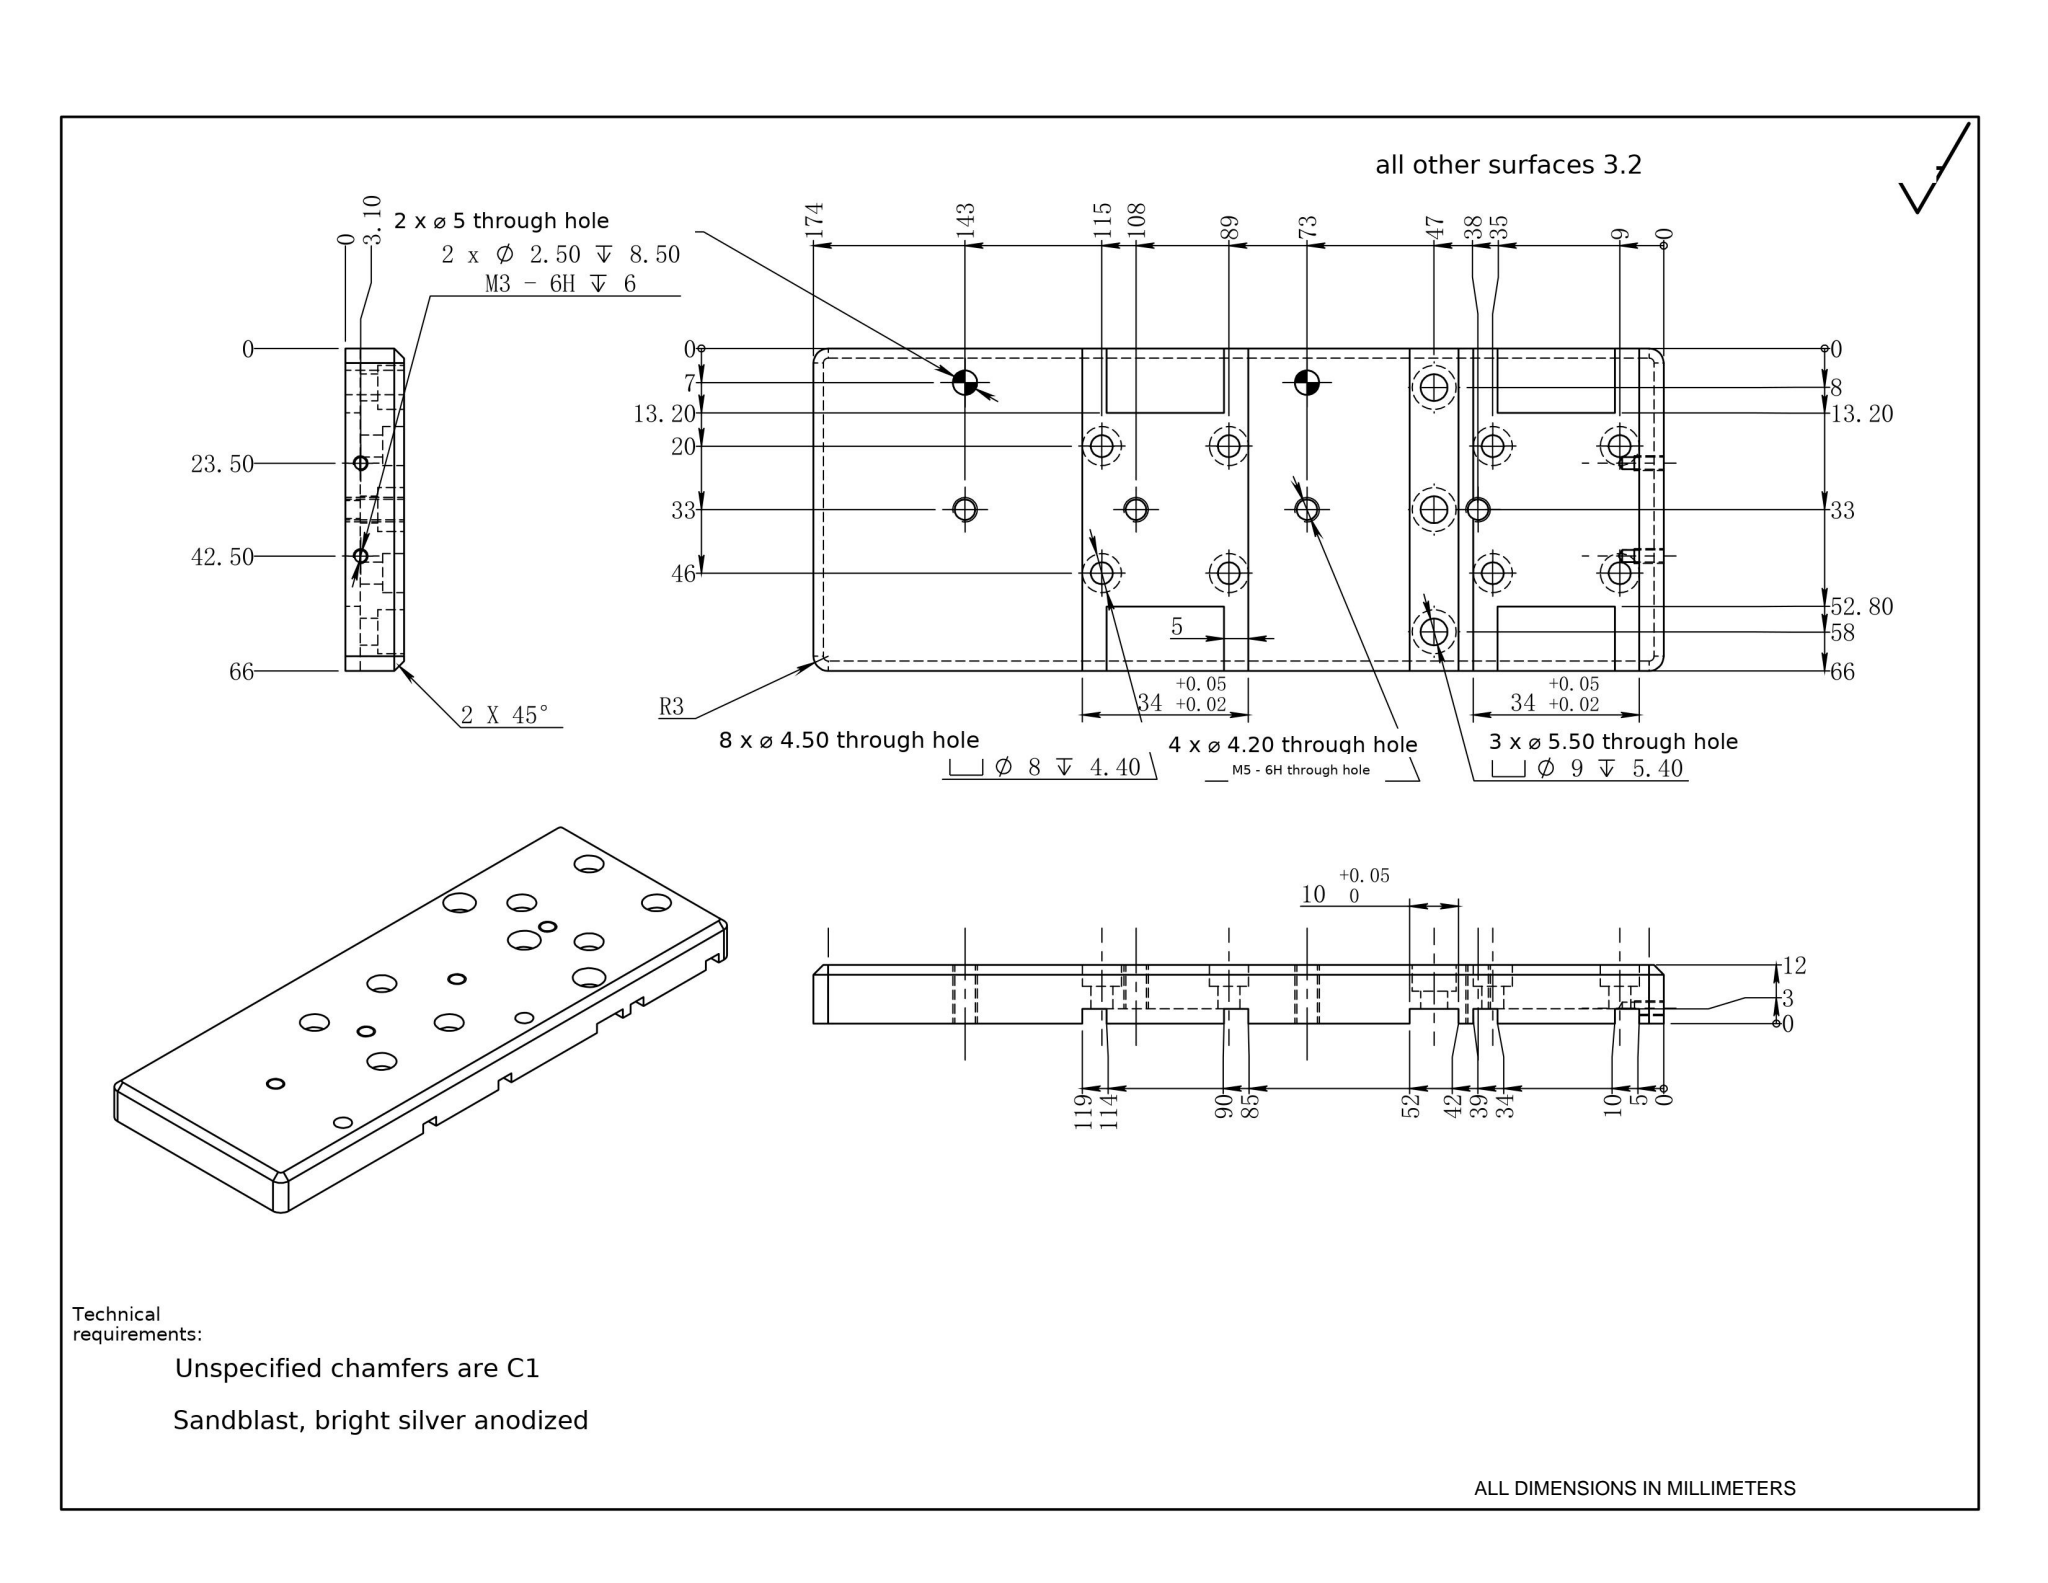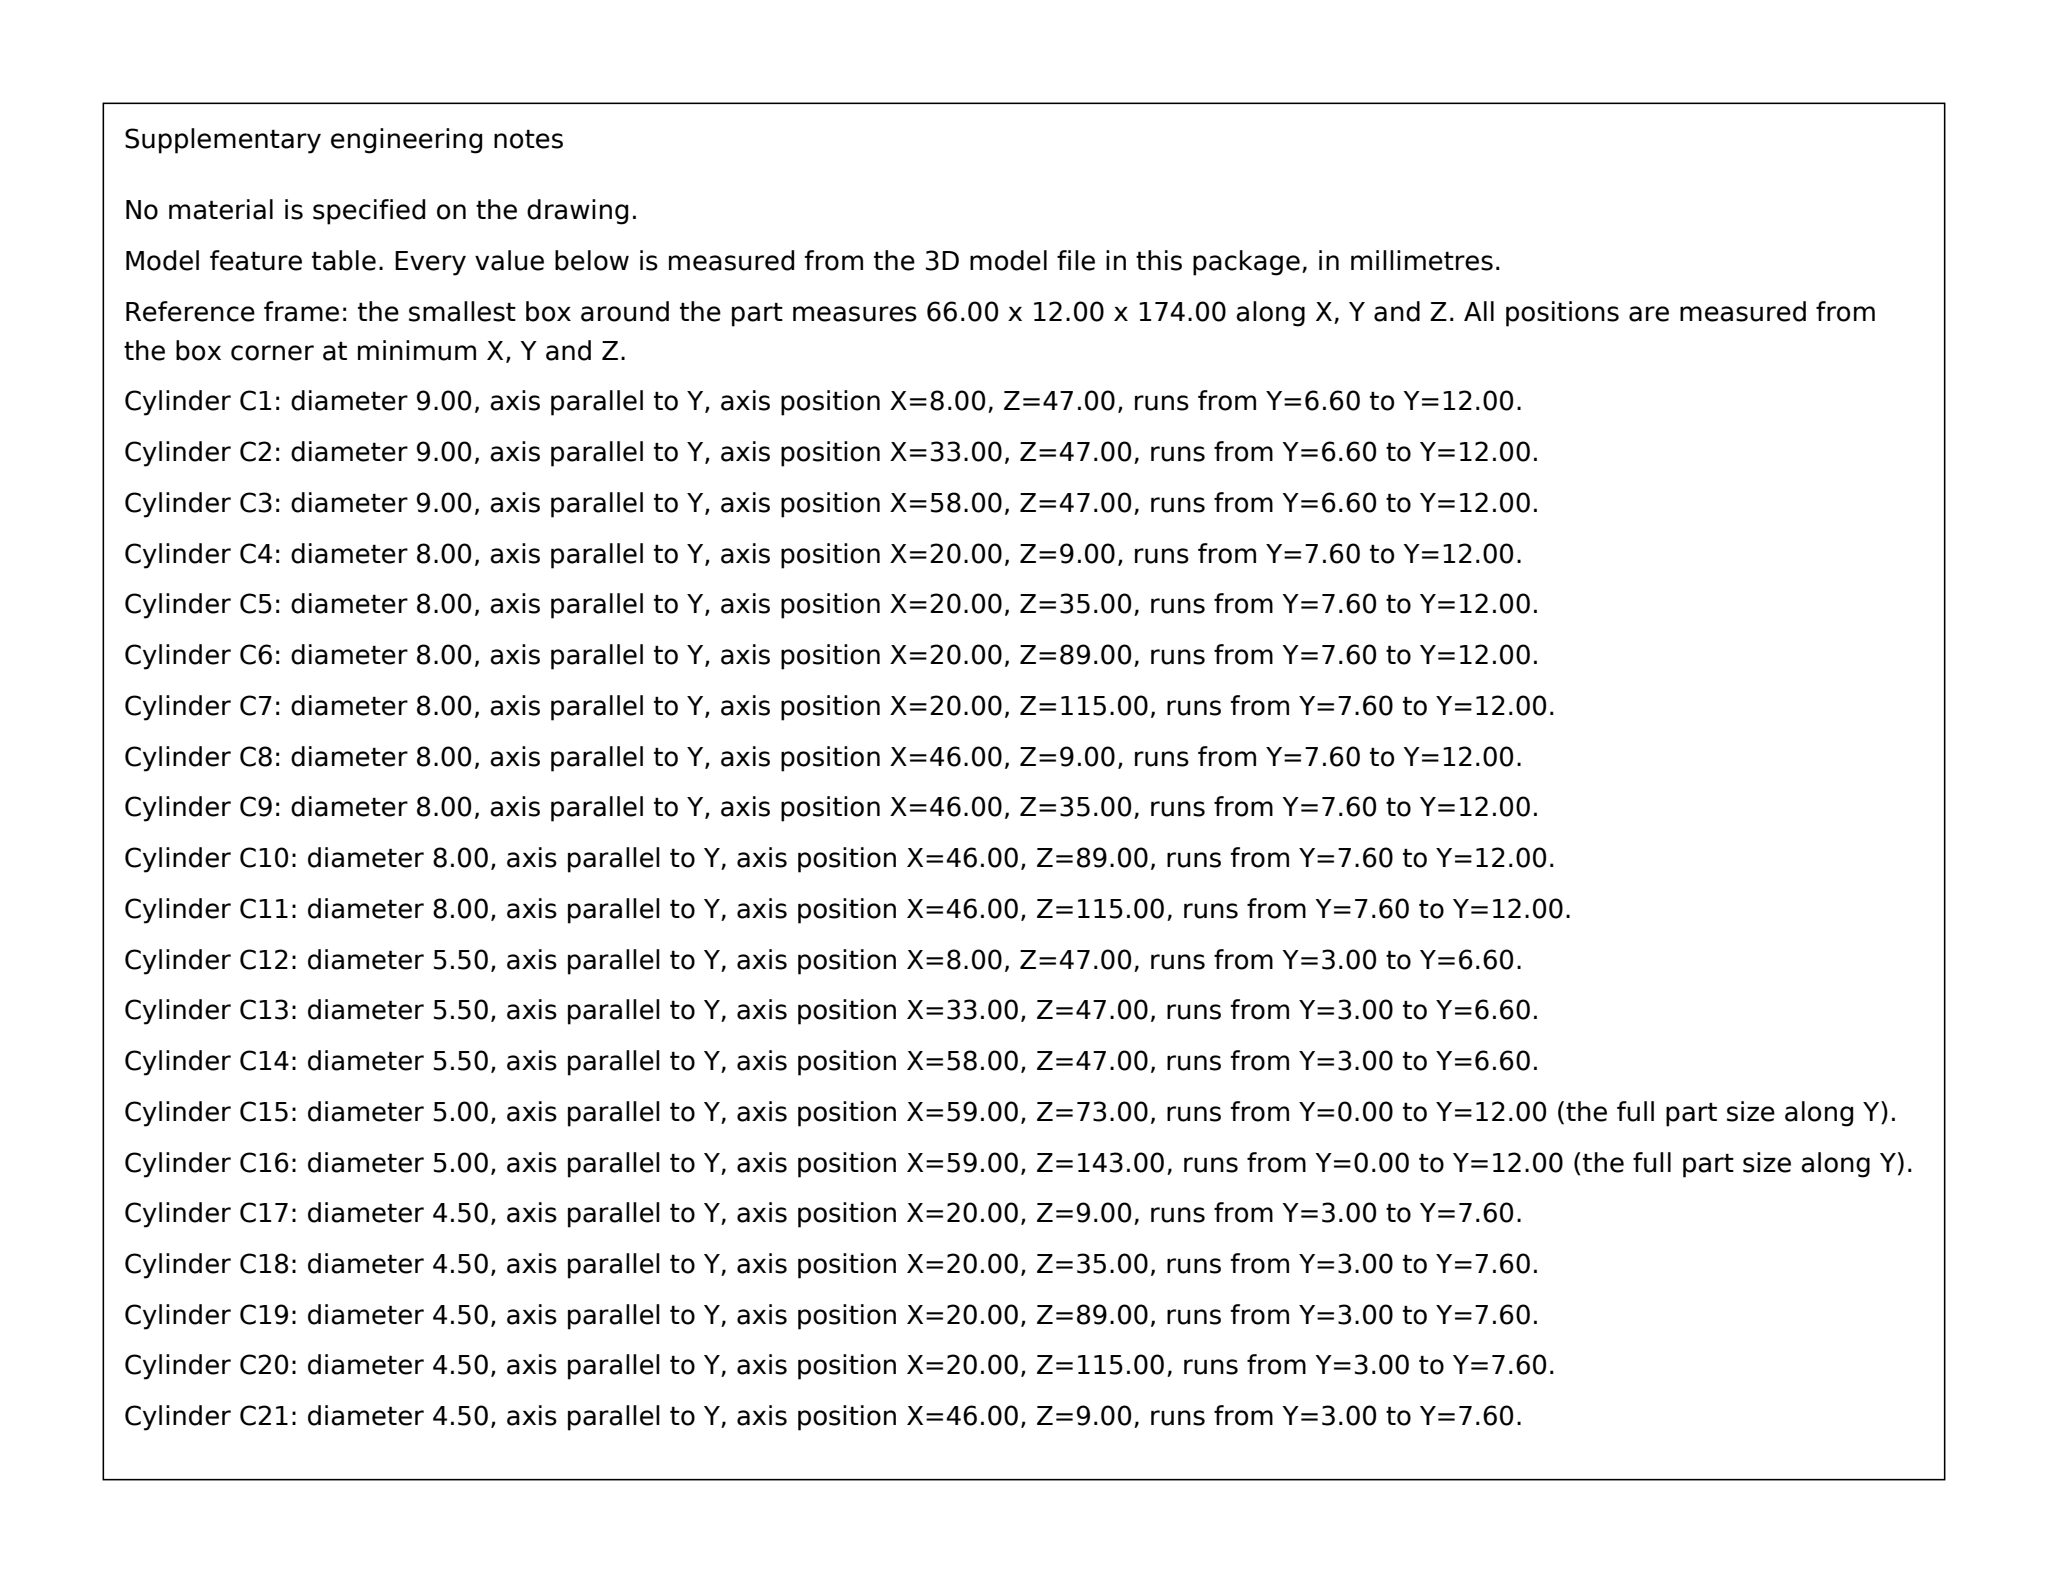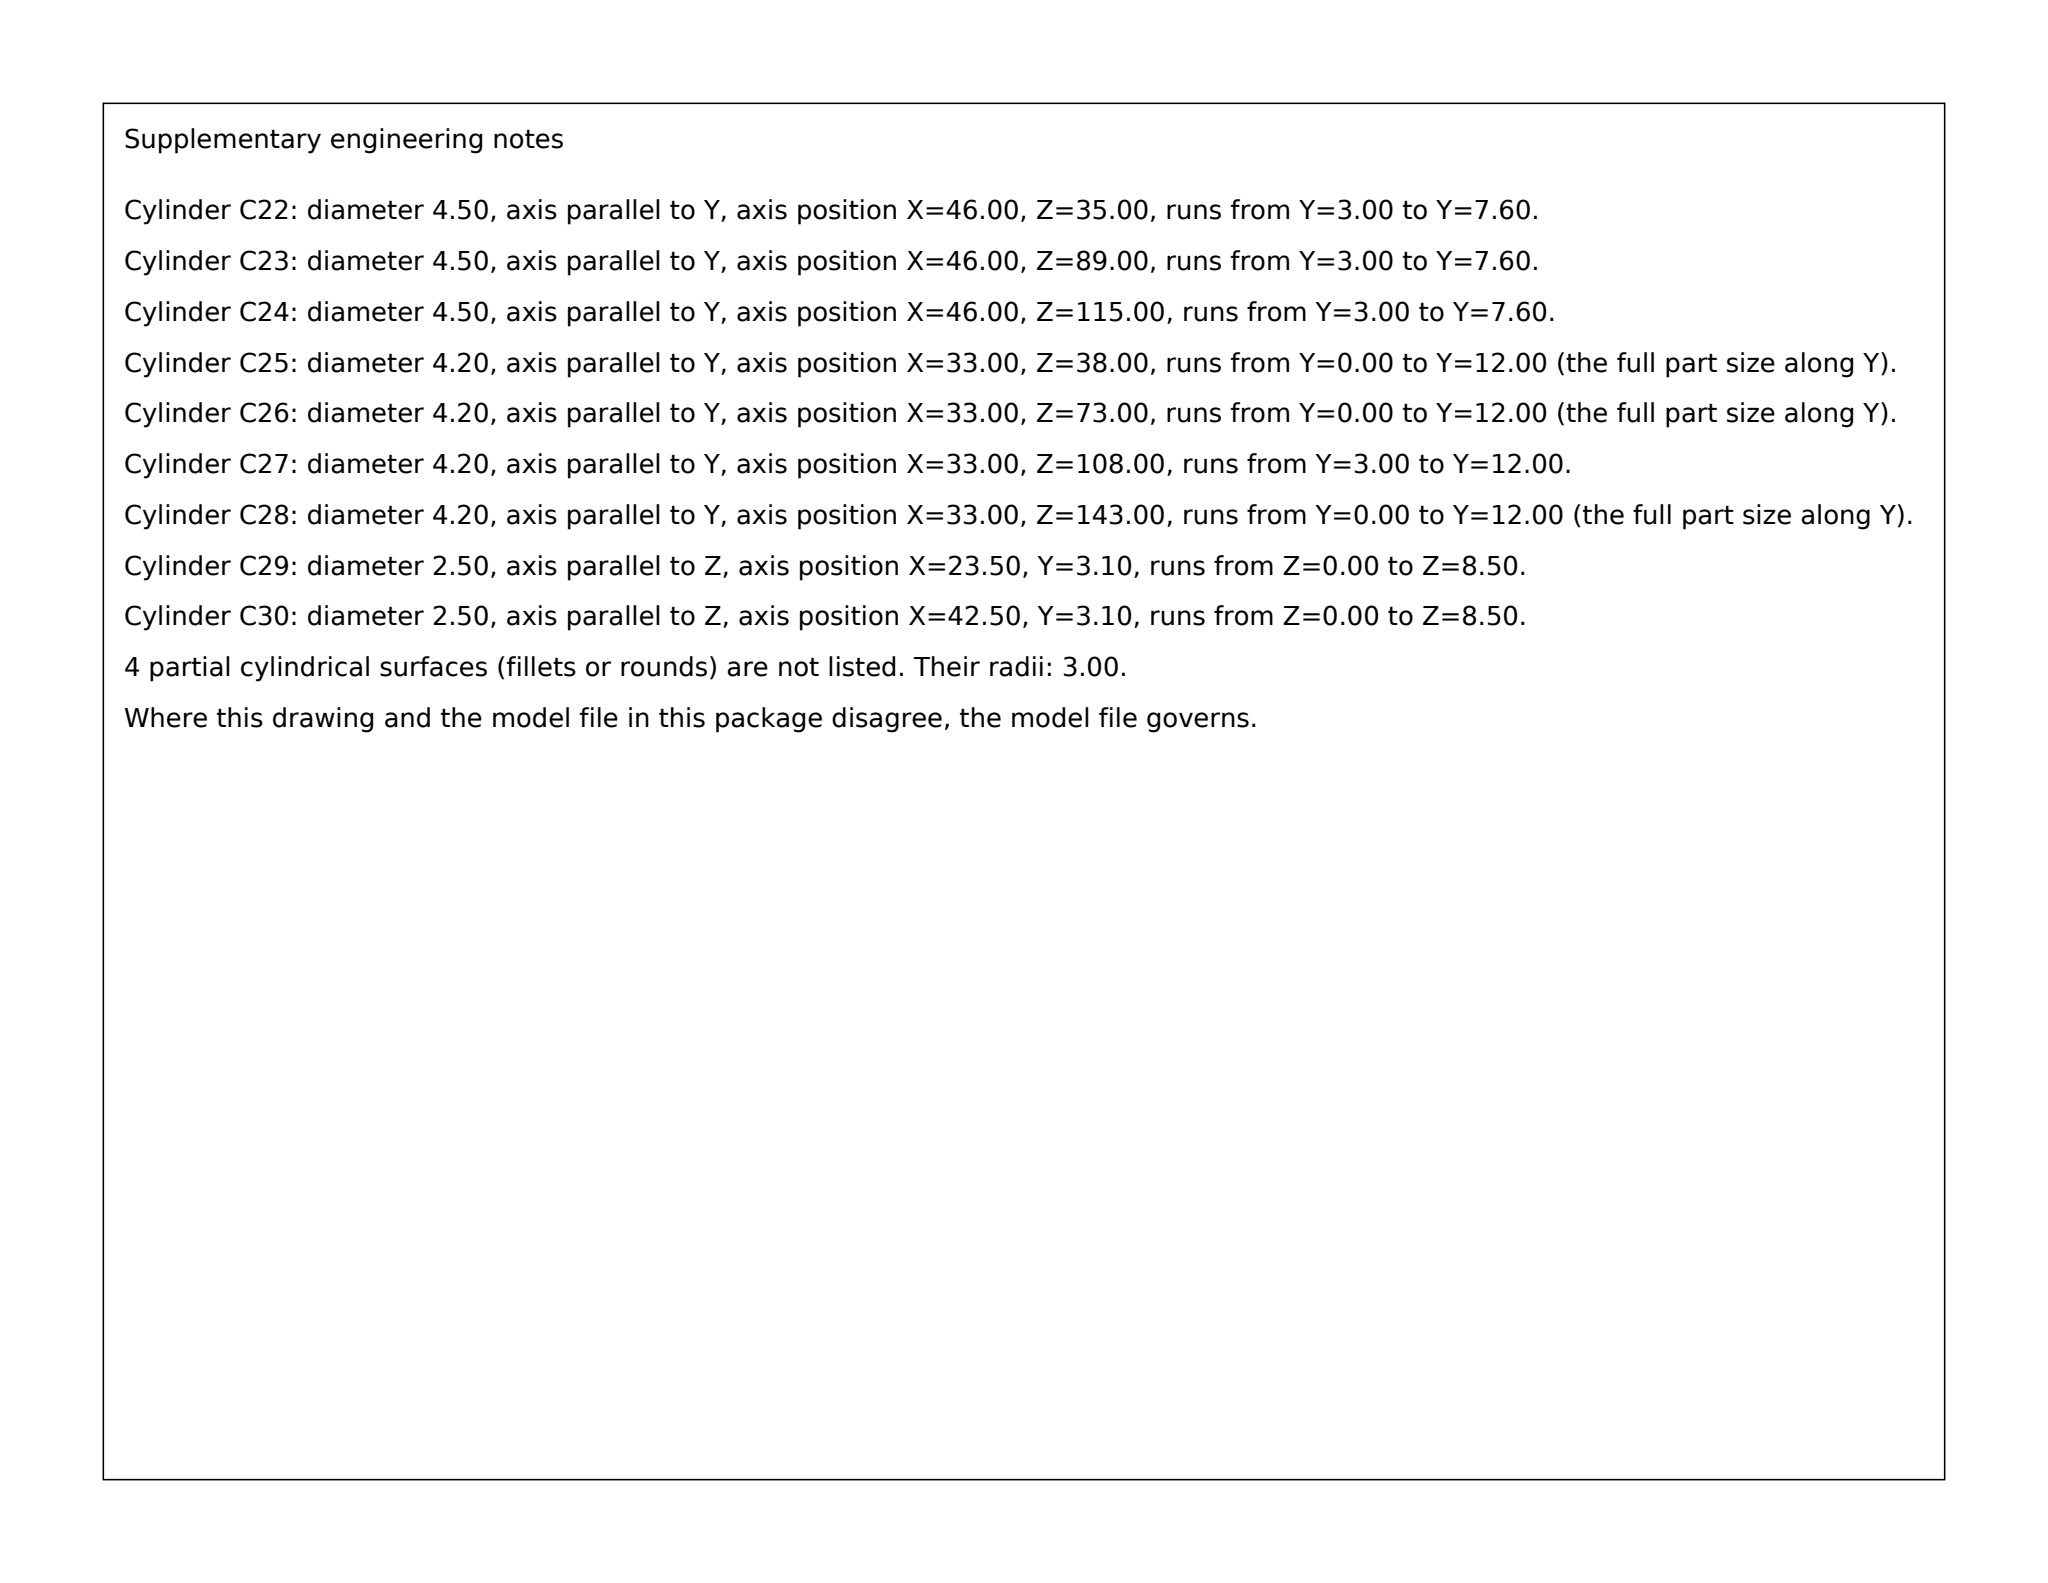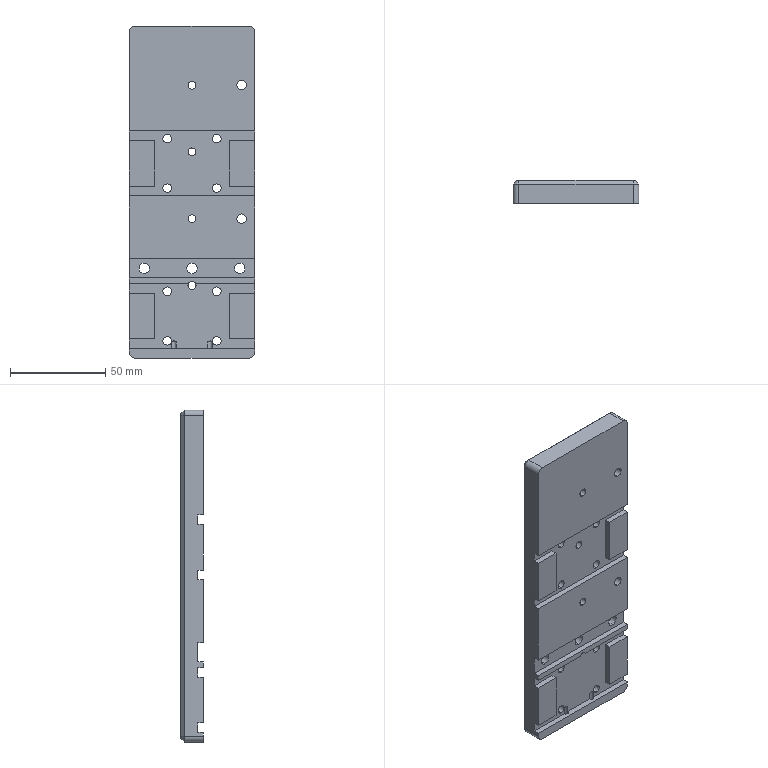Part | SolidWorks | mm | 1 solid | 122 faces | box 66 x 12 x 174 mm | volume 120359 mm3 | cylinder 64 | plane 50 | cone 8 | commonest cylinder face diameters 8 x16 4.5 x16 4.2 x8 9 x6 5.5 x6 2.5 x4 5 x4 6 x4
build123d program:
from build123d import *

# Parameters (mm, degrees)
SKETCH1_W                                       = 66
SKETCH1_H                                       = 174
BOSS_EXTRUDE1_DEPTH                             = 12
SKETCH2_W                                       = 66
SKETCH2_H                                       = 34
CUT_EXTRUDE1_DEPTH                              = 3
SKETCH3_W                                       = 66
SKETCH3_H                                       = 10
CUT_EXTRUDE2_DEPTH                              = 3
M5_HEX_SOCKET_HEAD_CAP_SCREW_CBORE1_D           = 5.5
M5_HEX_SOCKET_HEAD_CAP_SCREW_CBORE1_CBORE_D     = 9
M5_HEX_SOCKET_HEAD_CAP_SCREW_CBORE1_CBORE_DEPTH = 5.4
SKETCH7_W                                       = 13.2
SKETCH7_H                                       = 24
BOSS_EXTRUDE2_DEPTH                             = 3
M4_HEX_SOCKET_HEAD_CAP_SCREW_CBORE1_D           = 4.5
M4_HEX_SOCKET_HEAD_CAP_SCREW_CBORE1_CBORE_D     = 8
M4_HEX_SOCKET_HEAD_CAP_SCREW_CBORE1_CBORE_DEPTH = 4.4
M5_TAPPED_HOLE1_D                               = 4.2
F_5_0_5_DIAMETER_HOLE1_D                        = 5
FILLET1_R                                       = 3
CHAMFER1_SIZE                                   = 2
M3_TAPPED_HOLE1_D                               = 2.5
M3_TAPPED_HOLE1_DEPTH                           = 8.5
M3_TAPPED_HOLE1_TIP                             = 0.7511


with BuildPart() as part:
    # Sketch1 → Boss-Extrude1 (new body)
    with BuildSketch(Plane(origin=(0, 0, 0), x_dir=(1, 0, 0), z_dir=(0, 1, 0))):
        Rectangle(SKETCH1_W, SKETCH1_H)
    extrude(amount=BOSS_EXTRUDE1_DEPTH)

    # Sketch2 → Cut-Extrude1 (cut)
    with BuildSketch(Plane.XZ):
        with Locations((0, 15)):
            Rectangle(SKETCH2_W, SKETCH2_H)
        with Locations((0, -65)):
            Rectangle(SKETCH2_W, SKETCH2_H)
    extrude(amount=-CUT_EXTRUDE1_DEPTH, mode=Mode.SUBTRACT)

    # Sketch3 → Cut-Extrude2 (cut)
    with BuildSketch(Plane.XZ):
        with Locations((0, -40)):
            Rectangle(SKETCH3_W, SKETCH3_H)
    extrude(amount=-CUT_EXTRUDE2_DEPTH, mode=Mode.SUBTRACT)

    # M5 Hex Socket Head Cap Screw CBORE1 (through all)
    with Locations(Plane(origin=(0, 12, 0), x_dir=(1, 0, 0), z_dir=(0, 1, 0))):
        with Locations((-25, 40), (0, 40), (25, 40)):
            CounterBoreHole(M5_HEX_SOCKET_HEAD_CAP_SCREW_CBORE1_D / 2, M5_HEX_SOCKET_HEAD_CAP_SCREW_CBORE1_CBORE_D / 2, M5_HEX_SOCKET_HEAD_CAP_SCREW_CBORE1_CBORE_DEPTH)

    # Sketch7 → Boss-Extrude2 (add)
    with BuildSketch(Plane.XZ.offset(-3)):
        with Locations((-26.4, 15)):
            Rectangle(SKETCH7_W, SKETCH7_H)
        with Locations((26.4, 15)):
            Rectangle(SKETCH7_W, SKETCH7_H)
        with Locations((-26.4, -65)):
            Rectangle(SKETCH7_W, SKETCH7_H)
        with Locations((26.4, -65)):
            Rectangle(SKETCH7_W, SKETCH7_H)
    extrude(amount=BOSS_EXTRUDE2_DEPTH)

    # M4 Hex Socket Head Cap Screw CBORE1 (through all)
    with Locations(Plane(origin=(0, 12, 0), x_dir=(1, 0, 0), z_dir=(0, 1, 0))):
        with Locations((-13, 52), (13, 52), (13, 78), (-13, 78), (-13, -28), (13, -28), (13, -2), (-13, -2)):
            CounterBoreHole(M4_HEX_SOCKET_HEAD_CAP_SCREW_CBORE1_D / 2, M4_HEX_SOCKET_HEAD_CAP_SCREW_CBORE1_CBORE_D / 2, M4_HEX_SOCKET_HEAD_CAP_SCREW_CBORE1_CBORE_DEPTH)

    # M5 Tapped Hole1 (through all)
    with Locations(Plane(origin=(0, 12, 0), x_dir=(1, 0, 0), z_dir=(0, 1, 0))):
        with Locations((0, 49), (0, 14), (0, -21), (0, -56)):
            Hole(M5_TAPPED_HOLE1_D / 2)

    # 5.0 _5_ Diameter Hole1 (through all)
    with Locations(Plane(origin=(0, 0, 0), x_dir=(-1, 0, 0), z_dir=(0, -1, 0))):
        with Locations((-26, -56), (-26, 14)):
            Hole(F_5_0_5_DIAMETER_HOLE1_D / 2)

    # Fillet1
    fillet1_edges = [part.edges().sort_by_distance(p)[0] for p in [
        (33, 6, 87),
        (-33, 6, 87),
        (-33, 6, -87),
        (33, 6, -87),
    ]]
    fillet(fillet1_edges, radius=FILLET1_R)

    # Chamfer1
    chamfer1_edges = [part.edges().sort_by_distance(p)[0] for p in [
        (0, 12, -87),
        (33, 12, 0),
        (-33, 12, 0),
        (0, 12, 87),
        (-32.121, 12, 86.121),
        (32.121, 12, 86.121),
        (-32.121, 12, -86.121),
        (32.121, 12, -86.121),
    ]]
    chamfer(chamfer1_edges, length=CHAMFER1_SIZE)

    # M3 Tapped Hole1
    with Locations(Plane(origin=(0, 0, -87), x_dir=(-1, 0, 0), z_dir=(0, 0, -1))):
        with Locations((-9.5, 3.1), (9.5, 3.1)):
            Hole(M3_TAPPED_HOLE1_D / 2, depth=M3_TAPPED_HOLE1_DEPTH)
            with Locations((0, 0, -(M3_TAPPED_HOLE1_DEPTH + M3_TAPPED_HOLE1_TIP / 2))):  # 118° drill point
                Cone(0, M3_TAPPED_HOLE1_D / 2, M3_TAPPED_HOLE1_TIP, mode=Mode.SUBTRACT)


solid = part.part